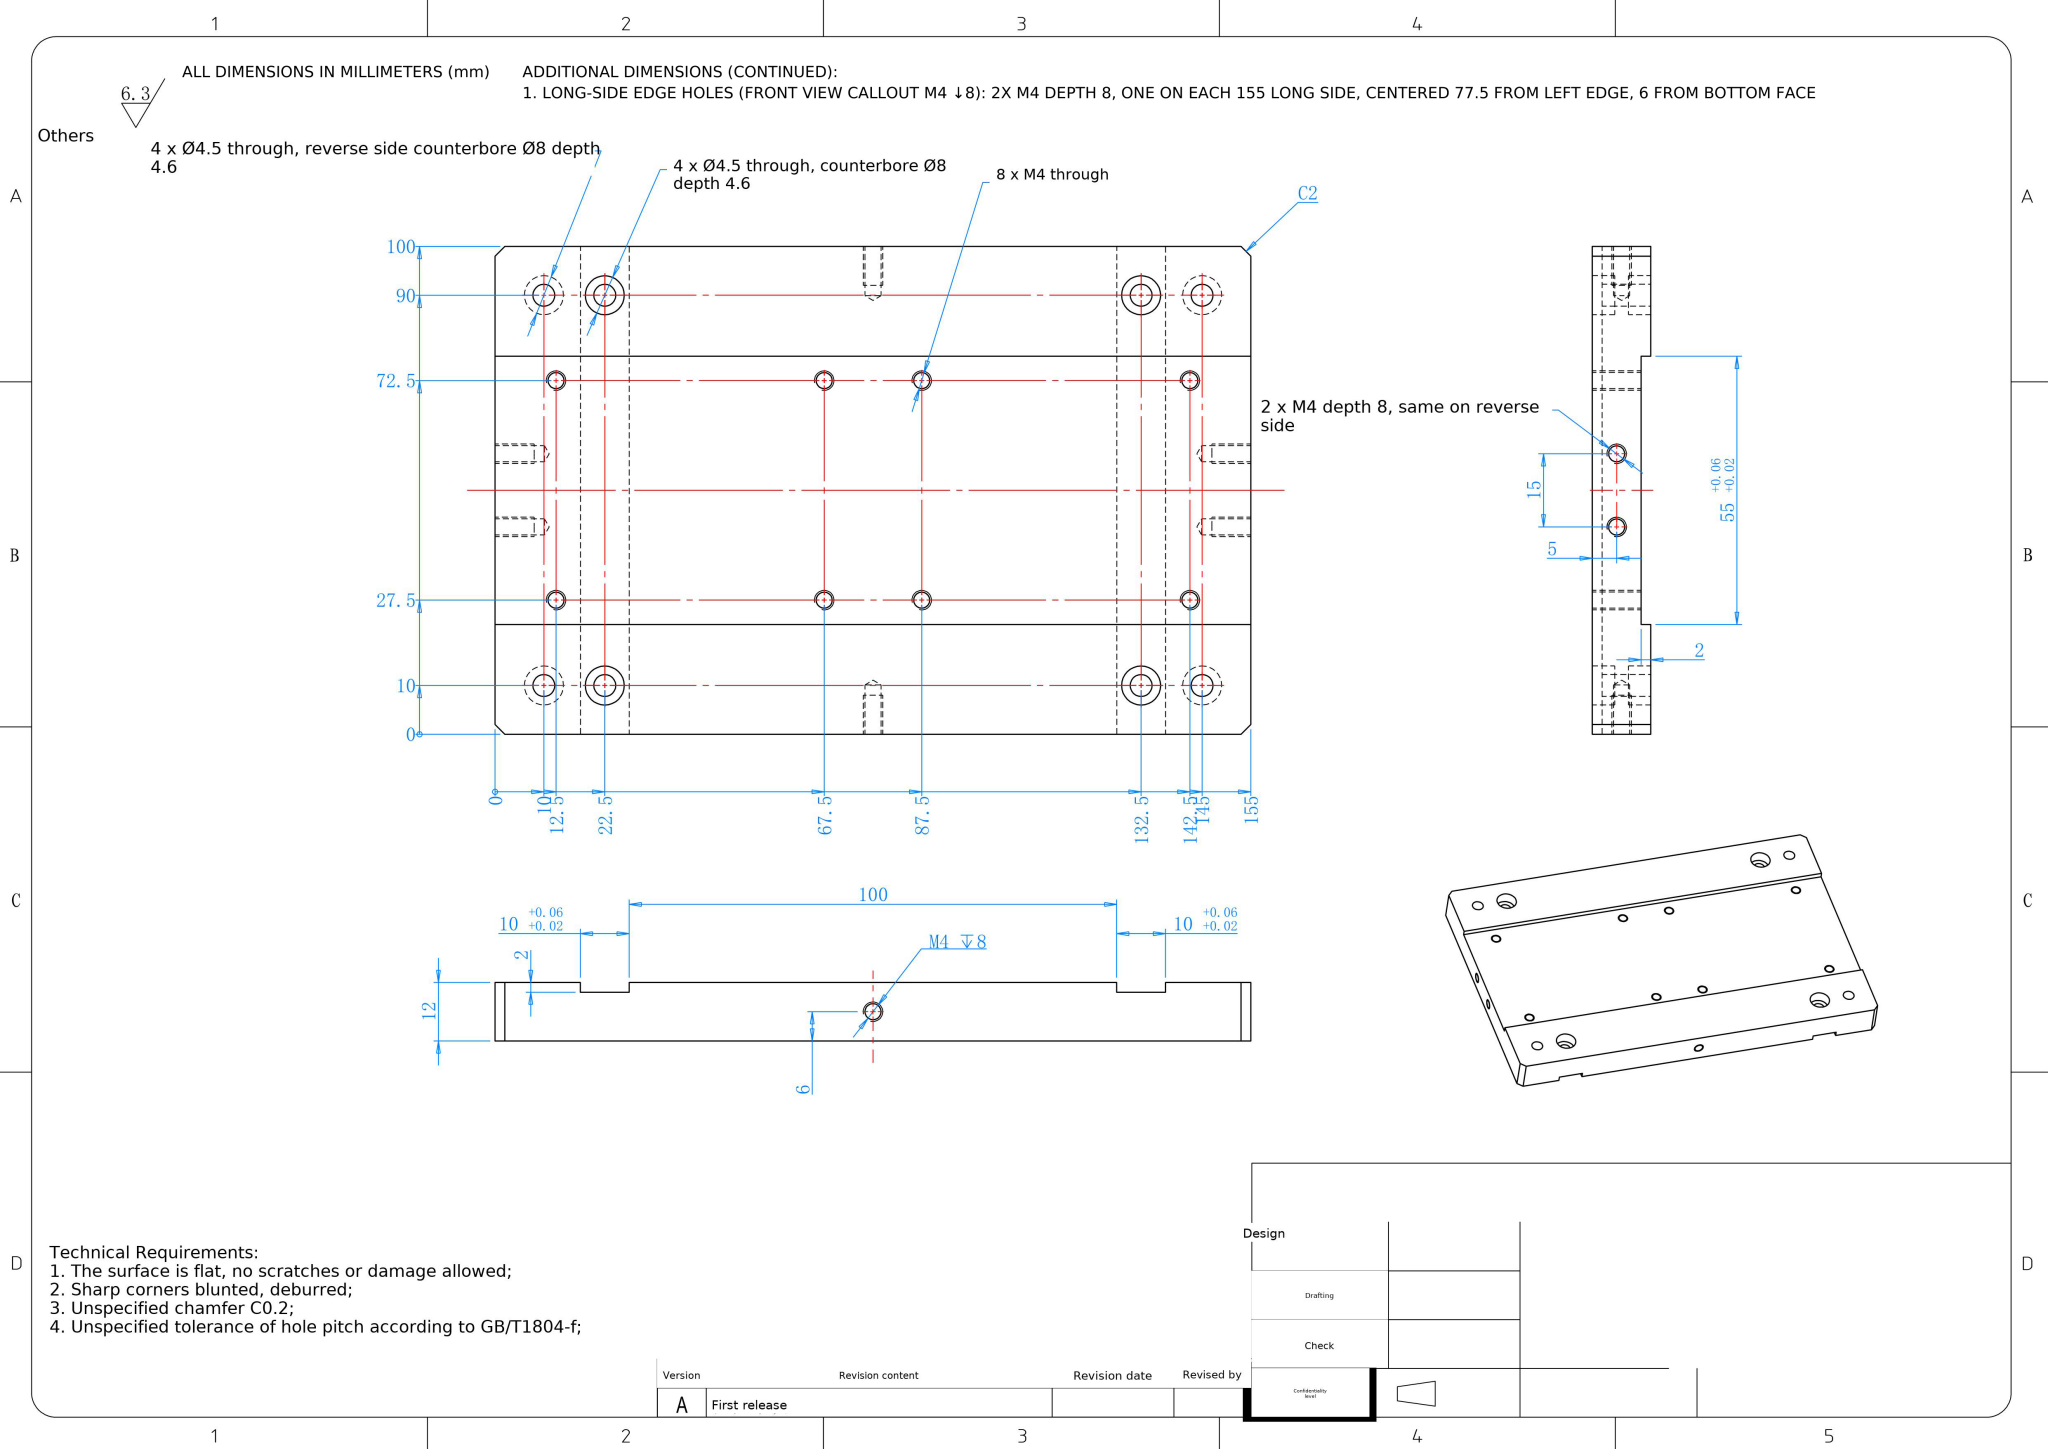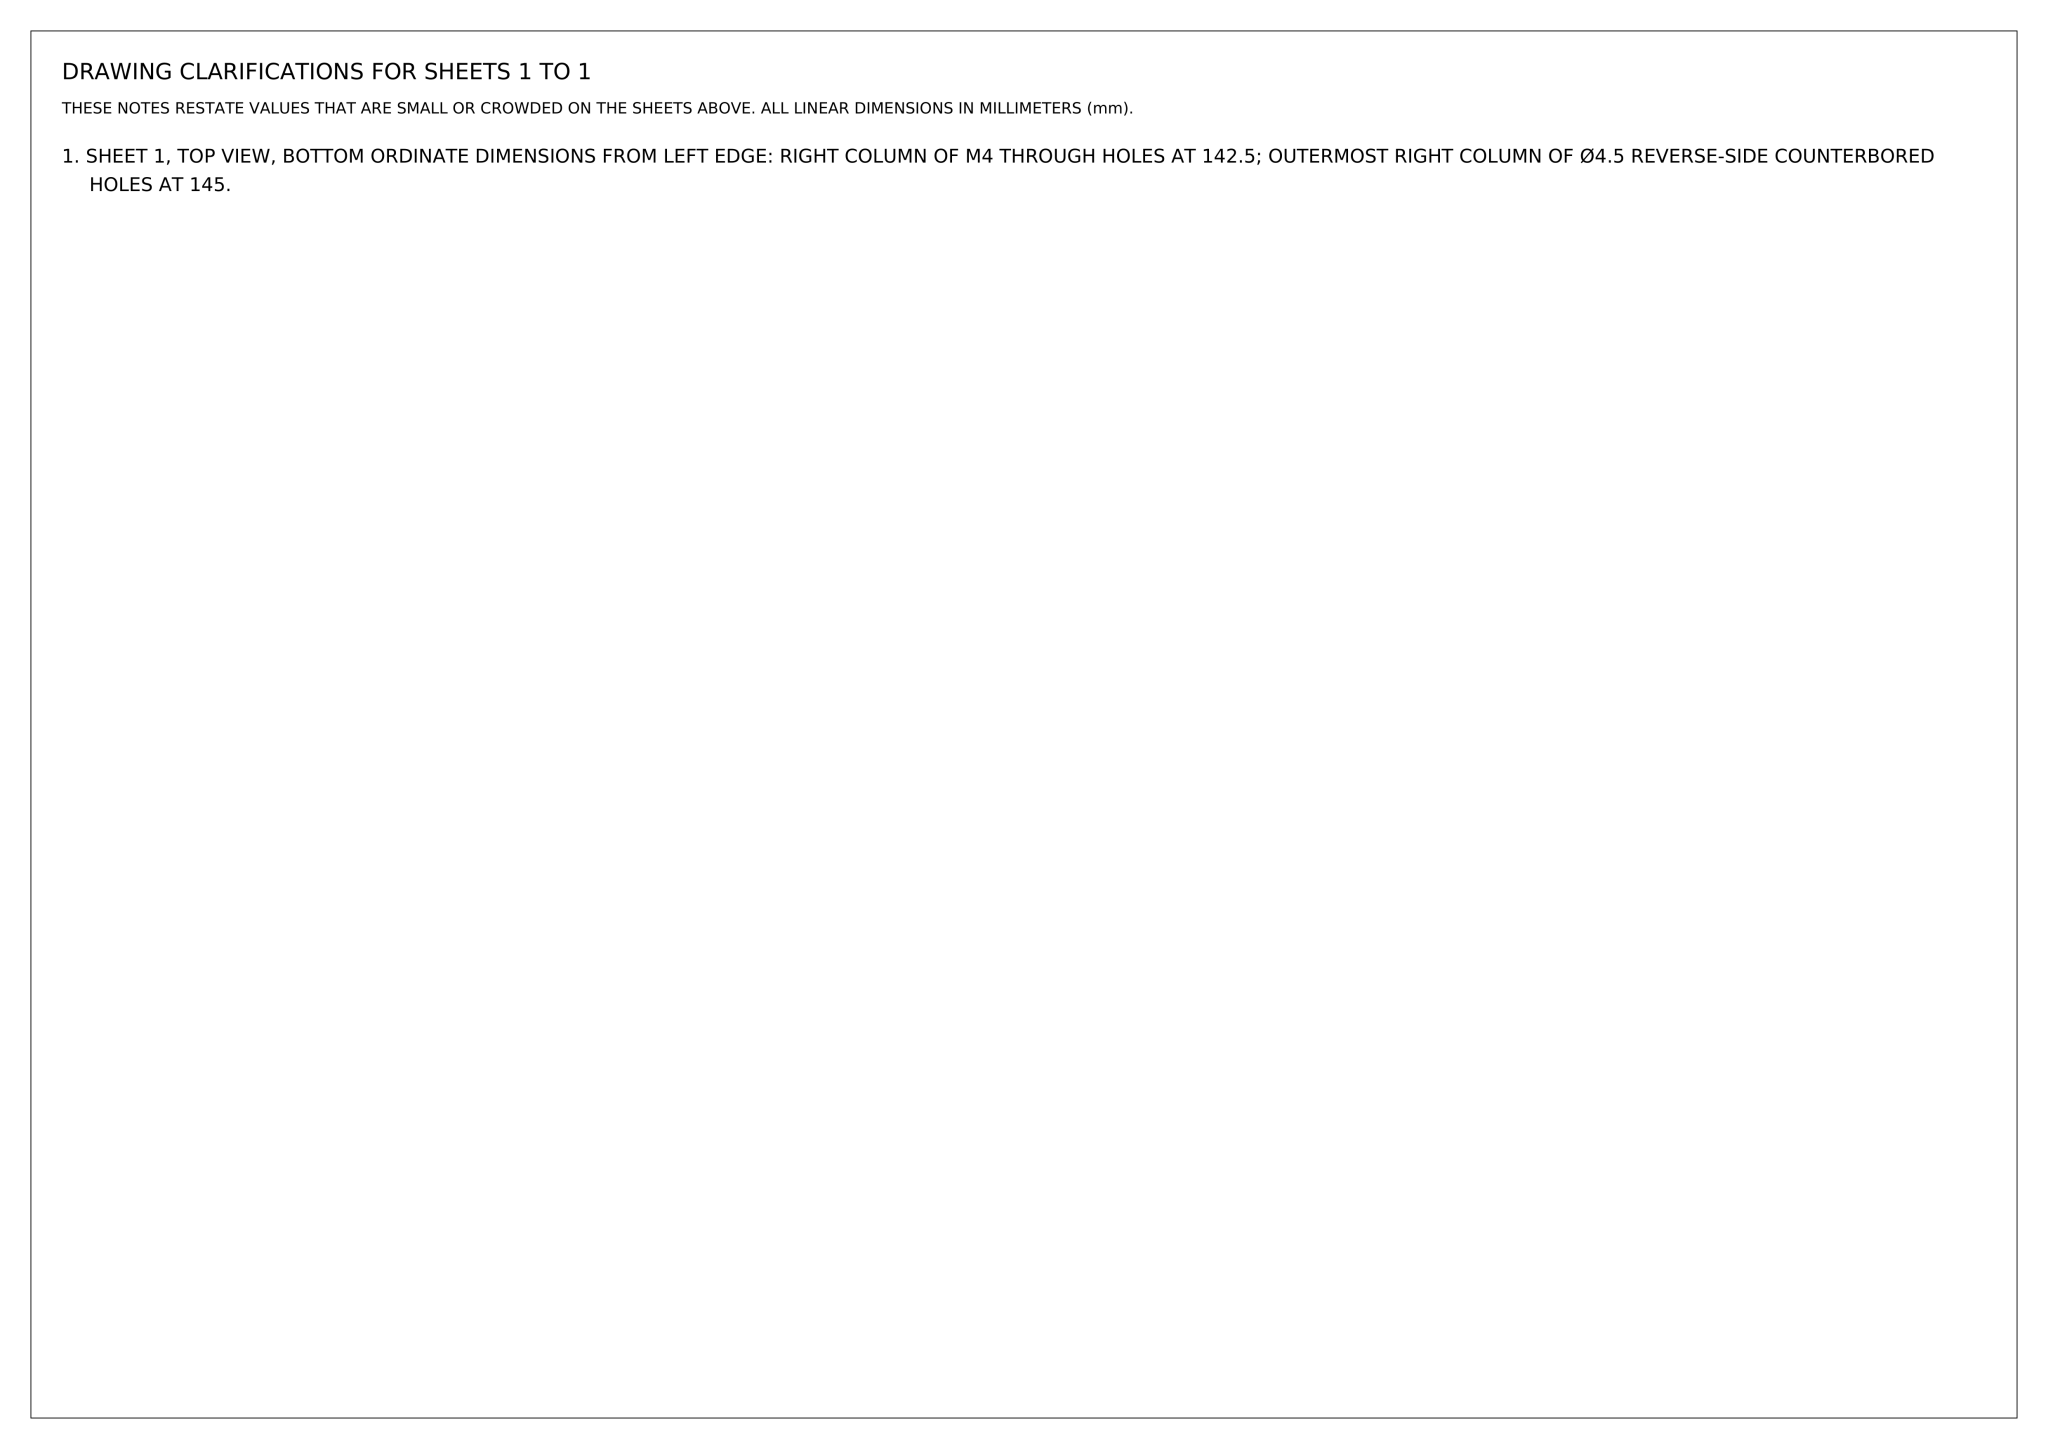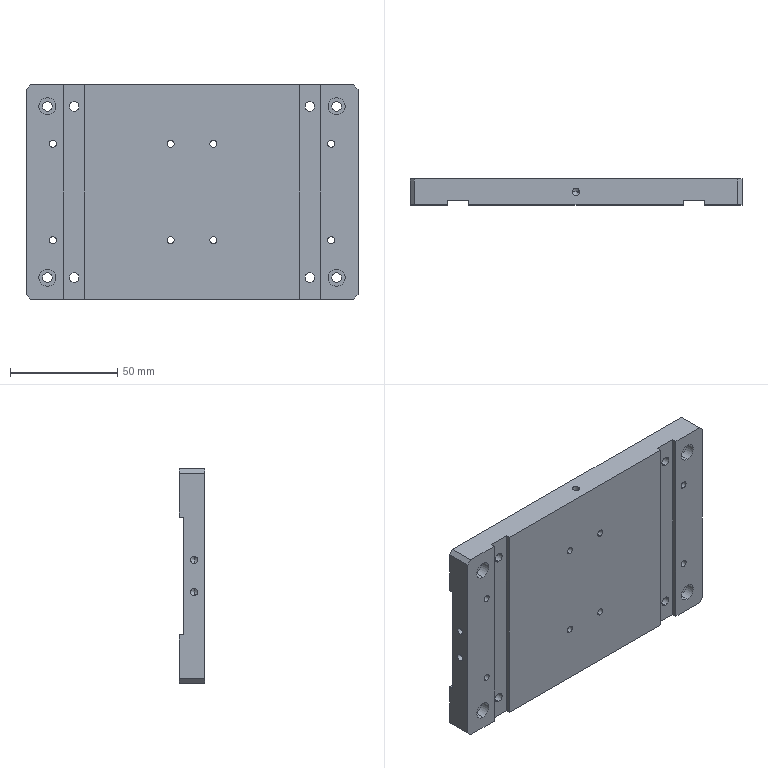Part | NX | mm | 1 solid | 102 faces | box 155 x 12 x 100 mm | volume 160970 mm3 | cylinder 60 | plane 30 | cone 12 | commonest cylinder face diameters 3.3 x28 8 x16 4.5 x16